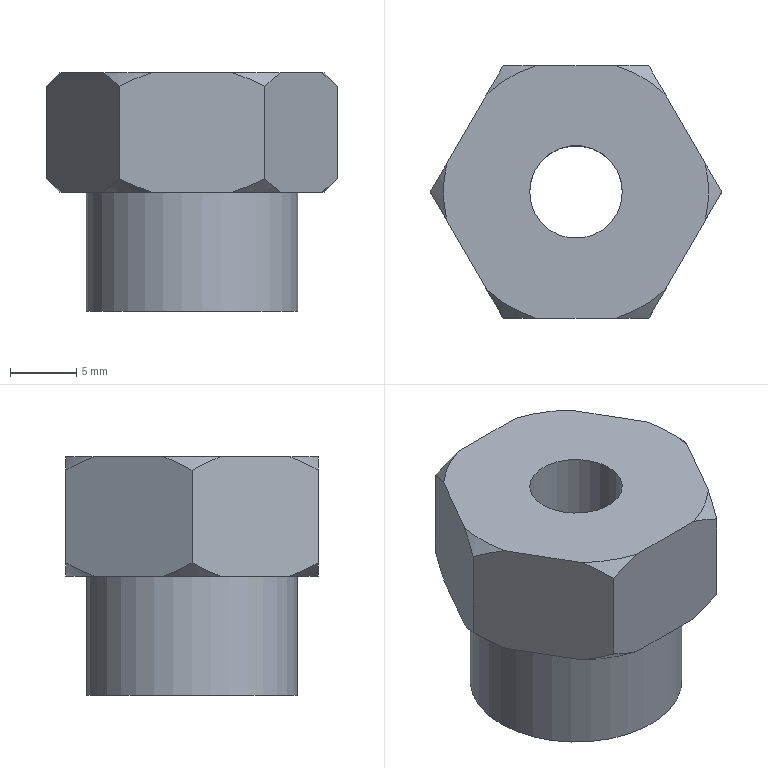Component | NX | GLAND | 1 solid | 23 faces | volume 3939 mm3 | cone 12 | plane 9 | cylinder 2 | commonest cylinder face diameters 16 x1 7 x1